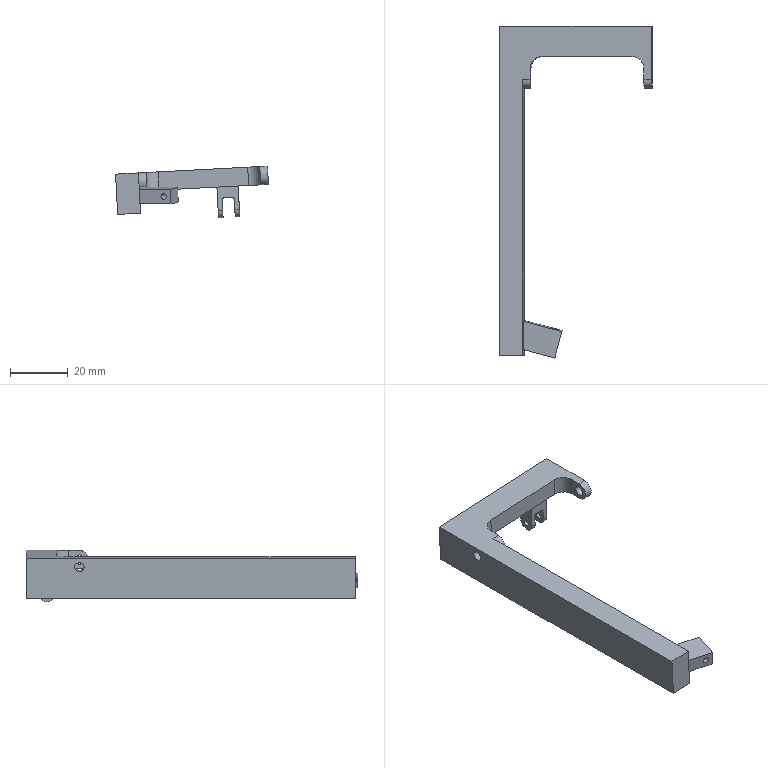Component | NX | MAIN_FRAME | 1 solid | 42 faces | volume 16759 mm3 | plane 23 | cylinder 16 | cone 3 | commonest cylinder face diameters 2.3 x3 5.292 x2 1.96 x2 8.467 x2 6.35 x2 3.3 x2 1.587 x2 1.97 x1